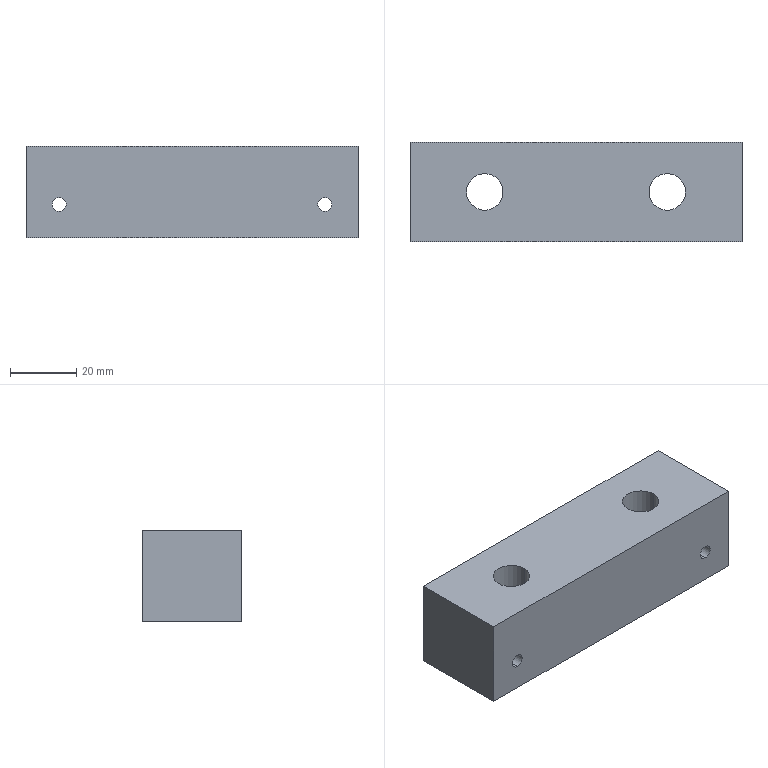Component | SolidWorks | RisingCylinderSeatPlate-1 | 1 solid | 20 faces | box 100 x 30 x 27.5 mm | volume 73803 mm3 | cylinder 12 | plane 8 | commonest cylinder face diameters 4.2 x4 17 x4 11 x4
build123d program:
from build123d import *

# Parameters (mm, degrees)
SKETCH1_W                                  = 100
SKETCH1_H                                  = 27.5
BOSS_EXTRUDE1_DEPTH                        = 30
M10_HEX_HEAD_BOLT_COUNTERBORE1_D           = 11
M10_HEX_HEAD_BOLT_COUNTERBORE1_CBORE_D     = 17
M10_HEX_HEAD_BOLT_COUNTERBORE1_CBORE_DEPTH = 10
M5_TAPPED_HOLE1_D                          = 4.2


with BuildPart() as part:
    # Sketch1 → Boss-Extrude1 (new body)
    with BuildSketch(Plane(origin=(0, 0, 0), x_dir=(1, 0, 0), z_dir=(0, 1, 0))):
        Rectangle(SKETCH1_W, SKETCH1_H)
    extrude(amount=BOSS_EXTRUDE1_DEPTH)

    # M10 Hex Head Bolt Counterbore1 (through all)
    with Locations(Plane(origin=(0, 0, -13.75), x_dir=(-1, 0, 0), z_dir=(0, 0, -1))):
        with Locations((-27.5, 15), (27.5, 15)):
            CounterBoreHole(M10_HEX_HEAD_BOLT_COUNTERBORE1_D / 2, M10_HEX_HEAD_BOLT_COUNTERBORE1_CBORE_D / 2, M10_HEX_HEAD_BOLT_COUNTERBORE1_CBORE_DEPTH)

    # M5 Tapped Hole1 (through all)
    with Locations(Plane(origin=(0, 30, 0), x_dir=(1, 0, 0), z_dir=(0, 1, 0))):
        with Locations((-40, 3.75), (40, 3.75)):
            Hole(M5_TAPPED_HOLE1_D / 2)


solid = part.part

# Placed as in the assembly
solid = solid.moved(Location((-29.507, -319.411, 406.75), (0, 0, 0)))
STEP:
#1=COLOUR_RGB('',0.7922,0.8196,0.9333);
#2=FILL_AREA_STYLE_COLOUR('',#1);
#3=FILL_AREA_STYLE('',(#2));
#4=SURFACE_STYLE_FILL_AREA(#3);
#5=SURFACE_SIDE_STYLE('',(#4));
#6=SURFACE_STYLE_USAGE(.BOTH.,#5);
#7=PRESENTATION_STYLE_ASSIGNMENT((#6));
#8=CARTESIAN_POINT('',(-2.736,-12.575,15.783));
#9=VERTEX_POINT('',#8);
#10=CARTESIAN_POINT('',(-2.736,-12.575,15.949));
#11=VERTEX_POINT('',#10);
#12=CARTESIAN_POINT('',(-2.736,-12.575,15.866));
#13=DIRECTION('',(0.,1.,0.));
#14=DIRECTION('',(0.,0.,1.));
#15=AXIS2_PLACEMENT_3D('',#12,#13,#14);
#16=CIRCLE('',#15,0.08268);
#17=EDGE_CURVE('',#9,#11,#16,.T.);
#18=ORIENTED_EDGE('',*,*,#17,.F.);
#19=CARTESIAN_POINT('',(-2.736,-11.394,15.783));
#20=VERTEX_POINT('',#19);
#21=CARTESIAN_POINT('',(-2.736,-11.394,15.783));
#22=DIRECTION('',(0.,1.,0.));
#23=VECTOR('',#22,39.37);
#24=LINE('',#21,#23);
#25=EDGE_CURVE('',#9,#20,#24,.T.);
#26=ORIENTED_EDGE('',*,*,#25,.T.);
#27=CARTESIAN_POINT('',(-2.736,-11.394,15.949));
#28=VERTEX_POINT('',#27);
#29=CARTESIAN_POINT('',(-2.736,-11.394,15.866));
#30=DIRECTION('',(0.,1.,0.));
#31=DIRECTION('',(0.,0.,1.));
#32=AXIS2_PLACEMENT_3D('',#29,#30,#31);
#33=CIRCLE('',#32,0.08268);
#34=EDGE_CURVE('',#20,#28,#33,.T.);
#35=ORIENTED_EDGE('',*,*,#34,.T.);
#36=CARTESIAN_POINT('',(-2.736,-11.394,15.949));
#37=DIRECTION('',(0.,1.,0.));
#38=VECTOR('',#37,39.37);
#39=LINE('',#36,#38);
#40=EDGE_CURVE('',#11,#28,#39,.T.);
#41=ORIENTED_EDGE('',*,*,#40,.F.);
#42=EDGE_LOOP('',(#18,#26,#35,#41));
#43=FACE_OUTER_BOUND('',#42,.T.);
#44=CARTESIAN_POINT('',(-2.736,-11.394,15.866));
#45=DIRECTION('',(0.,1.,0.));
#46=DIRECTION('',(0.,0.,1.));
#47=AXIS2_PLACEMENT_3D('',#44,#45,#46);
#48=CYLINDRICAL_SURFACE('',#47,0.08268);
#49=ADVANCED_FACE('',(#43),#48,.F.);
#50=CARTESIAN_POINT('',(0.4131,-12.575,15.783));
#51=VERTEX_POINT('',#50);
#52=CARTESIAN_POINT('',(0.4131,-12.575,15.949));
#53=VERTEX_POINT('',#52);
#54=CARTESIAN_POINT('',(0.4131,-12.575,15.866));
#55=DIRECTION('',(0.,1.,0.));
#56=DIRECTION('',(0.,0.,1.));
#57=AXIS2_PLACEMENT_3D('',#54,#55,#56);
#58=CIRCLE('',#57,0.08268);
#59=EDGE_CURVE('',#51,#53,#58,.T.);
#60=ORIENTED_EDGE('',*,*,#59,.F.);
#61=CARTESIAN_POINT('',(0.4131,-11.394,15.783));
#62=VERTEX_POINT('',#61);
#63=CARTESIAN_POINT('',(0.4131,-11.394,15.783));
#64=DIRECTION('',(0.,1.,0.));
#65=VECTOR('',#64,39.37);
#66=LINE('',#63,#65);
#67=EDGE_CURVE('',#51,#62,#66,.T.);
#68=ORIENTED_EDGE('',*,*,#67,.T.);
#69=CARTESIAN_POINT('',(0.4131,-11.394,15.949));
#70=VERTEX_POINT('',#69);
#71=CARTESIAN_POINT('',(0.4131,-11.394,15.866));
#72=DIRECTION('',(0.,1.,0.));
#73=DIRECTION('',(0.,0.,1.));
#74=AXIS2_PLACEMENT_3D('',#71,#72,#73);
#75=CIRCLE('',#74,0.08268);
#76=EDGE_CURVE('',#62,#70,#75,.T.);
#77=ORIENTED_EDGE('',*,*,#76,.T.);
#78=CARTESIAN_POINT('',(0.4131,-11.394,15.949));
#79=DIRECTION('',(0.,1.,0.));
#80=VECTOR('',#79,39.37);
#81=LINE('',#78,#80);
#82=EDGE_CURVE('',#53,#70,#81,.T.);
#83=ORIENTED_EDGE('',*,*,#82,.F.);
#84=EDGE_LOOP('',(#60,#68,#77,#83));
#85=FACE_OUTER_BOUND('',#84,.T.);
#86=CARTESIAN_POINT('',(0.4131,-11.394,15.866));
#87=DIRECTION('',(0.,1.,0.));
#88=DIRECTION('',(0.,0.,1.));
#89=AXIS2_PLACEMENT_3D('',#86,#87,#88);
#90=CYLINDRICAL_SURFACE('',#89,0.08268);
#91=ADVANCED_FACE('',(#85),#90,.F.);
#92=CARTESIAN_POINT('',(0.2556,-11.985,15.866));
#93=VERTEX_POINT('',#92);
#94=CARTESIAN_POINT('',(-0.4136,-11.985,15.866));
#95=VERTEX_POINT('',#94);
#96=CARTESIAN_POINT('',(-0.079,-11.985,15.866));
#97=DIRECTION('',(0.,0.,-1.));
#98=DIRECTION('',(-1.,0.,0.));
#99=AXIS2_PLACEMENT_3D('',#96,#97,#98);
#100=CIRCLE('',#99,0.3346);
#101=EDGE_CURVE('',#93,#95,#100,.T.);
#102=ORIENTED_EDGE('',*,*,#101,.F.);
#103=CARTESIAN_POINT('',(0.2556,-11.985,15.472));
#104=VERTEX_POINT('',#103);
#105=CARTESIAN_POINT('',(0.2556,-11.985,15.472));
#106=DIRECTION('',(0.,0.,-1.));
#107=VECTOR('',#106,39.37);
#108=LINE('',#105,#107);
#109=EDGE_CURVE('',#93,#104,#108,.T.);
#110=ORIENTED_EDGE('',*,*,#109,.T.);
#111=CARTESIAN_POINT('',(-0.4136,-11.985,15.472));
#112=VERTEX_POINT('',#111);
#113=CARTESIAN_POINT('',(-0.079,-11.985,15.472));
#114=DIRECTION('',(0.,0.,-1.));
#115=DIRECTION('',(-1.,0.,0.));
#116=AXIS2_PLACEMENT_3D('',#113,#114,#115);
#117=CIRCLE('',#116,0.3346);
#118=EDGE_CURVE('',#104,#112,#117,.T.);
#119=ORIENTED_EDGE('',*,*,#118,.T.);
#120=CARTESIAN_POINT('',(-0.4136,-11.985,15.472));
#121=DIRECTION('',(0.,0.,-1.));
#122=VECTOR('',#121,39.37);
#123=LINE('',#120,#122);
#124=EDGE_CURVE('',#95,#112,#123,.T.);
#125=ORIENTED_EDGE('',*,*,#124,.F.);
#126=EDGE_LOOP('',(#102,#110,#119,#125));
#127=FACE_OUTER_BOUND('',#126,.T.);
#128=CARTESIAN_POINT('',(-0.079,-11.985,15.472));
#129=DIRECTION('',(0.,0.,-1.));
#130=DIRECTION('',(-1.,0.,0.));
#131=AXIS2_PLACEMENT_3D('',#128,#129,#130);
#132=CYLINDRICAL_SURFACE('',#131,0.3346);
#133=ADVANCED_FACE('',(#127),#132,.F.);
#134=CARTESIAN_POINT('',(0.1375,-11.985,16.555));
#135=VERTEX_POINT('',#134);
#136=CARTESIAN_POINT('',(-0.2955,-11.985,16.555));
#137=VERTEX_POINT('',#136);
#138=CARTESIAN_POINT('',(-0.079,-11.985,16.555));
#139=DIRECTION('',(0.,0.,-1.));
#140=DIRECTION('',(-1.,0.,0.));
#141=AXIS2_PLACEMENT_3D('',#138,#139,#140);
#142=CIRCLE('',#141,0.2165);
#143=EDGE_CURVE('',#135,#137,#142,.T.);
#144=ORIENTED_EDGE('',*,*,#143,.F.);
#145=CARTESIAN_POINT('',(0.1375,-11.985,15.866));
#146=VERTEX_POINT('',#145);
#147=CARTESIAN_POINT('',(0.1375,-11.985,15.472));
#148=DIRECTION('',(0.,0.,-1.));
#149=VECTOR('',#148,39.37);
#150=LINE('',#147,#149);
#151=EDGE_CURVE('',#135,#146,#150,.T.);
#152=ORIENTED_EDGE('',*,*,#151,.T.);
#153=CARTESIAN_POINT('',(-0.2955,-11.985,15.866));
#154=VERTEX_POINT('',#153);
#155=CARTESIAN_POINT('',(-0.079,-11.985,15.866));
#156=DIRECTION('',(0.,0.,-1.));
#157=DIRECTION('',(-1.,0.,0.));
#158=AXIS2_PLACEMENT_3D('',#155,#156,#157);
#159=CIRCLE('',#158,0.2165);
#160=EDGE_CURVE('',#146,#154,#159,.T.);
#161=ORIENTED_EDGE('',*,*,#160,.T.);
#162=CARTESIAN_POINT('',(-0.2955,-11.985,15.472));
#163=DIRECTION('',(0.,0.,-1.));
#164=VECTOR('',#163,39.37);
#165=LINE('',#162,#164);
#166=EDGE_CURVE('',#137,#154,#165,.T.);
#167=ORIENTED_EDGE('',*,*,#166,.F.);
#168=EDGE_LOOP('',(#144,#152,#161,#167));
#169=FACE_OUTER_BOUND('',#168,.T.);
#170=CARTESIAN_POINT('',(-0.079,-11.985,15.472));
#171=DIRECTION('',(0.,0.,-1.));
#172=DIRECTION('',(-1.,0.,0.));
#173=AXIS2_PLACEMENT_3D('',#170,#171,#172);
#174=CYLINDRICAL_SURFACE('',#173,0.2165);
#175=ADVANCED_FACE('',(#169),#174,.F.);
#176=CARTESIAN_POINT('',(-1.91,-11.985,15.866));
#177=VERTEX_POINT('',#176);
#178=CARTESIAN_POINT('',(-2.579,-11.985,15.866));
#179=VERTEX_POINT('',#178);
#180=CARTESIAN_POINT('',(-2.244,-11.985,15.866));
#181=DIRECTION('',(0.,0.,-1.));
#182=DIRECTION('',(-1.,0.,0.));
#183=AXIS2_PLACEMENT_3D('',#180,#181,#182);
#184=CIRCLE('',#183,0.3346);
#185=EDGE_CURVE('',#177,#179,#184,.T.);
#186=ORIENTED_EDGE('',*,*,#185,.F.);
#187=CARTESIAN_POINT('',(-1.91,-11.985,15.472));
#188=VERTEX_POINT('',#187);
#189=CARTESIAN_POINT('',(-1.91,-11.985,15.472));
#190=DIRECTION('',(0.,0.,-1.));
#191=VECTOR('',#190,39.37);
#192=LINE('',#189,#191);
#193=EDGE_CURVE('',#177,#188,#192,.T.);
#194=ORIENTED_EDGE('',*,*,#193,.T.);
#195=CARTESIAN_POINT('',(-2.579,-11.985,15.472));
#196=VERTEX_POINT('',#195);
#197=CARTESIAN_POINT('',(-2.244,-11.985,15.472));
#198=DIRECTION('',(0.,0.,-1.));
#199=DIRECTION('',(-1.,0.,0.));
#200=AXIS2_PLACEMENT_3D('',#197,#198,#199);
#201=CIRCLE('',#200,0.3346);
#202=EDGE_CURVE('',#188,#196,#201,.T.);
#203=ORIENTED_EDGE('',*,*,#202,.T.);
#204=CARTESIAN_POINT('',(-2.579,-11.985,15.472));
#205=DIRECTION('',(0.,0.,-1.));
#206=VECTOR('',#205,39.37);
#207=LINE('',#204,#206);
#208=EDGE_CURVE('',#179,#196,#207,.T.);
#209=ORIENTED_EDGE('',*,*,#208,.F.);
#210=EDGE_LOOP('',(#186,#194,#203,#209));
#211=FACE_OUTER_BOUND('',#210,.T.);
#212=CARTESIAN_POINT('',(-2.244,-11.985,15.472));
#213=DIRECTION('',(0.,0.,-1.));
#214=DIRECTION('',(-1.,0.,0.));
#215=AXIS2_PLACEMENT_3D('',#212,#213,#214);
#216=CYLINDRICAL_SURFACE('',#215,0.3346);
#217=ADVANCED_FACE('',(#211),#216,.F.);
#218=CARTESIAN_POINT('',(-2.028,-11.985,16.555));
#219=VERTEX_POINT('',#218);
#220=CARTESIAN_POINT('',(-2.461,-11.985,16.555));
#221=VERTEX_POINT('',#220);
#222=CARTESIAN_POINT('',(-2.244,-11.985,16.555));
#223=DIRECTION('',(0.,0.,-1.));
#224=DIRECTION('',(-1.,0.,0.));
#225=AXIS2_PLACEMENT_3D('',#222,#223,#224);
#226=CIRCLE('',#225,0.2165);
#227=EDGE_CURVE('',#219,#221,#226,.T.);
#228=ORIENTED_EDGE('',*,*,#227,.F.);
#229=CARTESIAN_POINT('',(-2.028,-11.985,15.866));
#230=VERTEX_POINT('',#229);
#231=CARTESIAN_POINT('',(-2.028,-11.985,15.472));
#232=DIRECTION('',(0.,0.,-1.));
#233=VECTOR('',#232,39.37);
#234=LINE('',#231,#233);
#235=EDGE_CURVE('',#219,#230,#234,.T.);
#236=ORIENTED_EDGE('',*,*,#235,.T.);
#237=CARTESIAN_POINT('',(-2.461,-11.985,15.866));
#238=VERTEX_POINT('',#237);
#239=CARTESIAN_POINT('',(-2.244,-11.985,15.866));
#240=DIRECTION('',(0.,0.,-1.));
#241=DIRECTION('',(-1.,0.,0.));
#242=AXIS2_PLACEMENT_3D('',#239,#240,#241);
#243=CIRCLE('',#242,0.2165);
#244=EDGE_CURVE('',#230,#238,#243,.T.);
#245=ORIENTED_EDGE('',*,*,#244,.T.);
#246=CARTESIAN_POINT('',(-2.461,-11.985,15.472));
#247=DIRECTION('',(0.,0.,-1.));
#248=VECTOR('',#247,39.37);
#249=LINE('',#246,#248);
#250=EDGE_CURVE('',#221,#238,#249,.T.);
#251=ORIENTED_EDGE('',*,*,#250,.F.);
#252=EDGE_LOOP('',(#228,#236,#245,#251));
#253=FACE_OUTER_BOUND('',#252,.T.);
#254=CARTESIAN_POINT('',(-2.244,-11.985,15.472));
#255=DIRECTION('',(0.,0.,-1.));
#256=DIRECTION('',(-1.,0.,0.));
#257=AXIS2_PLACEMENT_3D('',#254,#255,#256);
#258=CYLINDRICAL_SURFACE('',#257,0.2165);
#259=ADVANCED_FACE('',(#253),#258,.F.);
#260=CARTESIAN_POINT('',(-3.13,-12.575,15.472));
#261=VERTEX_POINT('',#260);
#262=CARTESIAN_POINT('',(-3.13,-12.575,16.555));
#263=VERTEX_POINT('',#262);
#264=CARTESIAN_POINT('',(-3.13,-12.575,16.555));
#265=DIRECTION('',(0.,0.,1.));
#266=VECTOR('',#265,39.37);
#267=LINE('',#264,#266);
#268=EDGE_CURVE('',#261,#263,#267,.T.);
#269=ORIENTED_EDGE('',*,*,#268,.T.);
#270=CARTESIAN_POINT('',(-3.13,-11.394,16.555));
#271=VERTEX_POINT('',#270);
#272=CARTESIAN_POINT('',(-3.13,-11.394,16.555));
#273=DIRECTION('',(0.,-1.,0.));
#274=VECTOR('',#273,39.37);
#275=LINE('',#272,#274);
#276=EDGE_CURVE('',#271,#263,#275,.T.);
#277=ORIENTED_EDGE('',*,*,#276,.F.);
#278=CARTESIAN_POINT('',(-3.13,-11.394,15.472));
#279=VERTEX_POINT('',#278);
#280=CARTESIAN_POINT('',(-3.13,-11.394,16.555));
#281=DIRECTION('',(0.,0.,1.));
#282=VECTOR('',#281,39.37);
#283=LINE('',#280,#282);
#284=EDGE_CURVE('',#279,#271,#283,.T.);
#285=ORIENTED_EDGE('',*,*,#284,.F.);
#286=CARTESIAN_POINT('',(-3.13,-11.394,15.472));
#287=DIRECTION('',(0.,-1.,0.));
#288=VECTOR('',#287,39.37);
#289=LINE('',#286,#288);
#290=EDGE_CURVE('',#279,#261,#289,.T.);
#291=ORIENTED_EDGE('',*,*,#290,.T.);
#292=EDGE_LOOP('',(#269,#277,#285,#291));
#293=FACE_OUTER_BOUND('',#292,.T.);
#294=CARTESIAN_POINT('',(-3.13,-11.394,16.555));
#295=DIRECTION('',(1.,0.,0.));
#296=DIRECTION('',(0.,0.,-1.));
#297=AXIS2_PLACEMENT_3D('',#294,#295,#296);
#298=PLANE('',#297);
#299=ADVANCED_FACE('',(#293),#298,.F.);
#300=CARTESIAN_POINT('',(-0.079,-11.985,16.555));
#301=DIRECTION('',(0.,0.,-1.));
#302=DIRECTION('',(-1.,0.,0.));
#303=AXIS2_PLACEMENT_3D('',#300,#301,#302);
#304=CIRCLE('',#303,0.2165);
#305=EDGE_CURVE('',#137,#135,#304,.T.);
#306=ORIENTED_EDGE('',*,*,#305,.T.);
#307=ORIENTED_EDGE('',*,*,#143,.T.);
#308=EDGE_LOOP('',(#306,#307));
#309=FACE_BOUND('',#308,.T.);
#310=CARTESIAN_POINT('',(-2.244,-11.985,16.555));
#311=DIRECTION('',(0.,0.,-1.));
#312=DIRECTION('',(-1.,0.,0.));
#313=AXIS2_PLACEMENT_3D('',#310,#311,#312);
#314=CIRCLE('',#313,0.2165);
#315=EDGE_CURVE('',#221,#219,#314,.T.);
#316=ORIENTED_EDGE('',*,*,#315,.T.);
#317=ORIENTED_EDGE('',*,*,#227,.T.);
#318=EDGE_LOOP('',(#316,#317));
#319=FACE_BOUND('',#318,.T.);
#320=CARTESIAN_POINT('',(0.8068,-12.575,16.555));
#321=VERTEX_POINT('',#320);
#322=CARTESIAN_POINT('',(0.8068,-12.575,16.555));
#323=DIRECTION('',(1.,0.,-0.));
#324=VECTOR('',#323,39.37);
#325=LINE('',#322,#324);
#326=EDGE_CURVE('',#263,#321,#325,.T.);
#327=ORIENTED_EDGE('',*,*,#326,.T.);
#328=CARTESIAN_POINT('',(0.8068,-11.394,16.555));
#329=VERTEX_POINT('',#328);
#330=CARTESIAN_POINT('',(0.8068,-11.394,16.555));
#331=DIRECTION('',(0.,-1.,0.));
#332=VECTOR('',#331,39.37);
#333=LINE('',#330,#332);
#334=EDGE_CURVE('',#329,#321,#333,.T.);
#335=ORIENTED_EDGE('',*,*,#334,.F.);
#336=CARTESIAN_POINT('',(0.8068,-11.394,16.555));
#337=DIRECTION('',(1.,0.,-0.));
#338=VECTOR('',#337,39.37);
#339=LINE('',#336,#338);
#340=EDGE_CURVE('',#271,#329,#339,.T.);
#341=ORIENTED_EDGE('',*,*,#340,.F.);
#342=ORIENTED_EDGE('',*,*,#276,.T.);
#343=EDGE_LOOP('',(#327,#335,#341,#342));
#344=FACE_OUTER_BOUND('',#343,.T.);
#345=CARTESIAN_POINT('',(0.8068,-11.394,16.555));
#346=DIRECTION('',(-0.,0.,-1.));
#347=DIRECTION('',(-1.,0.,0.));
#348=AXIS2_PLACEMENT_3D('',#345,#346,#347);
#349=PLANE('',#348);
#350=ADVANCED_FACE('',(#309,#319,#344),#349,.F.);
#351=CARTESIAN_POINT('',(0.8068,-12.575,15.472));
#352=VERTEX_POINT('',#351);
#353=CARTESIAN_POINT('',(0.8068,-12.575,16.555));
#354=DIRECTION('',(0.,0.,-1.));
#355=VECTOR('',#354,39.37);
#356=LINE('',#353,#355);
#357=EDGE_CURVE('',#321,#352,#356,.T.);
#358=ORIENTED_EDGE('',*,*,#357,.T.);
#359=CARTESIAN_POINT('',(0.8068,-11.394,15.472));
#360=VERTEX_POINT('',#359);
#361=CARTESIAN_POINT('',(0.8068,-11.394,15.472));
#362=DIRECTION('',(0.,-1.,0.));
#363=VECTOR('',#362,39.37);
#364=LINE('',#361,#363);
#365=EDGE_CURVE('',#360,#352,#364,.T.);
#366=ORIENTED_EDGE('',*,*,#365,.F.);
#367=CARTESIAN_POINT('',(0.8068,-11.394,16.555));
#368=DIRECTION('',(0.,0.,-1.));
#369=VECTOR('',#368,39.37);
#370=LINE('',#367,#369);
#371=EDGE_CURVE('',#329,#360,#370,.T.);
#372=ORIENTED_EDGE('',*,*,#371,.F.);
#373=ORIENTED_EDGE('',*,*,#334,.T.);
#374=EDGE_LOOP('',(#358,#366,#372,#373));
#375=FACE_OUTER_BOUND('',#374,.T.);
#376=CARTESIAN_POINT('',(0.8068,-11.394,16.555));
#377=DIRECTION('',(-1.,0.,0.));
#378=DIRECTION('',(0.,0.,1.));
#379=AXIS2_PLACEMENT_3D('',#376,#377,#378);
#380=PLANE('',#379);
#381=ADVANCED_FACE('',(#375),#380,.F.);
#382=CARTESIAN_POINT('',(-0.079,-11.985,15.472));
#383=DIRECTION('',(0.,0.,-1.));
#384=DIRECTION('',(-1.,0.,0.));
#385=AXIS2_PLACEMENT_3D('',#382,#383,#384);
#386=CIRCLE('',#385,0.3346);
#387=EDGE_CURVE('',#112,#104,#386,.T.);
#388=ORIENTED_EDGE('',*,*,#387,.F.);
#389=ORIENTED_EDGE('',*,*,#118,.F.);
#390=EDGE_LOOP('',(#388,#389));
#391=FACE_BOUND('',#390,.T.);
#392=CARTESIAN_POINT('',(-2.244,-11.985,15.472));
#393=DIRECTION('',(0.,0.,-1.));
#394=DIRECTION('',(-1.,0.,0.));
#395=AXIS2_PLACEMENT_3D('',#392,#393,#394);
#396=CIRCLE('',#395,0.3346);
#397=EDGE_CURVE('',#196,#188,#396,.T.);
#398=ORIENTED_EDGE('',*,*,#397,.F.);
#399=ORIENTED_EDGE('',*,*,#202,.F.);
#400=EDGE_LOOP('',(#398,#399));
#401=FACE_BOUND('',#400,.T.);
#402=CARTESIAN_POINT('',(0.8068,-12.575,15.472));
#403=DIRECTION('',(-1.,0.,0.));
#404=VECTOR('',#403,39.37);
#405=LINE('',#402,#404);
#406=EDGE_CURVE('',#352,#261,#405,.T.);
#407=ORIENTED_EDGE('',*,*,#406,.T.);
#408=ORIENTED_EDGE('',*,*,#290,.F.);
#409=CARTESIAN_POINT('',(0.8068,-11.394,15.472));
#410=DIRECTION('',(-1.,0.,0.));
#411=VECTOR('',#410,39.37);
#412=LINE('',#409,#411);
#413=EDGE_CURVE('',#360,#279,#412,.T.);
#414=ORIENTED_EDGE('',*,*,#413,.F.);
#415=ORIENTED_EDGE('',*,*,#365,.T.);
#416=EDGE_LOOP('',(#407,#408,#414,#415));
#417=FACE_OUTER_BOUND('',#416,.T.);
#418=CARTESIAN_POINT('',(0.8068,-11.394,15.472));
#419=DIRECTION('',(0.,0.,1.));
#420=DIRECTION('',(1.,0.,-0.));
#421=AXIS2_PLACEMENT_3D('',#418,#419,#420);
#422=PLANE('',#421);
#423=ADVANCED_FACE('',(#391,#401,#417),#422,.F.);
#424=CARTESIAN_POINT('',(-2.736,-11.394,15.866));
#425=DIRECTION('',(0.,1.,0.));
#426=DIRECTION('',(0.,0.,1.));
#427=AXIS2_PLACEMENT_3D('',#424,#425,#426);
#428=CIRCLE('',#427,0.08268);
#429=EDGE_CURVE('',#28,#20,#428,.T.);
#430=ORIENTED_EDGE('',*,*,#429,.F.);
#431=ORIENTED_EDGE('',*,*,#34,.F.);
#432=EDGE_LOOP('',(#430,#431));
#433=FACE_BOUND('',#432,.T.);
#434=CARTESIAN_POINT('',(0.4131,-11.394,15.866));
#435=DIRECTION('',(0.,1.,0.));
#436=DIRECTION('',(0.,0.,1.));
#437=AXIS2_PLACEMENT_3D('',#434,#435,#436);
#438=CIRCLE('',#437,0.08268);
#439=EDGE_CURVE('',#70,#62,#438,.T.);
#440=ORIENTED_EDGE('',*,*,#439,.F.);
#441=ORIENTED_EDGE('',*,*,#76,.F.);
#442=EDGE_LOOP('',(#440,#441));
#443=FACE_BOUND('',#442,.T.);
#444=ORIENTED_EDGE('',*,*,#284,.T.);
#445=ORIENTED_EDGE('',*,*,#340,.T.);
#446=ORIENTED_EDGE('',*,*,#371,.T.);
#447=ORIENTED_EDGE('',*,*,#413,.T.);
#448=EDGE_LOOP('',(#444,#445,#446,#447));
#449=FACE_OUTER_BOUND('',#448,.T.);
#450=CARTESIAN_POINT('',(-1.162,-11.394,16.014));
#451=DIRECTION('',(0.,1.,0.));
#452=DIRECTION('',(0.,0.,1.));
#453=AXIS2_PLACEMENT_3D('',#450,#451,#452);
#454=PLANE('',#453);
#455=ADVANCED_FACE('',(#433,#443,#449),#454,.T.);
#456=CARTESIAN_POINT('',(-2.736,-12.575,15.866));
#457=DIRECTION('',(0.,1.,0.));
#458=DIRECTION('',(0.,0.,1.));
#459=AXIS2_PLACEMENT_3D('',#456,#457,#458);
#460=CIRCLE('',#459,0.08268);
#461=EDGE_CURVE('',#11,#9,#460,.T.);
#462=ORIENTED_EDGE('',*,*,#461,.T.);
#463=ORIENTED_EDGE('',*,*,#17,.T.);
#464=EDGE_LOOP('',(#462,#463));
#465=FACE_BOUND('',#464,.T.);
#466=CARTESIAN_POINT('',(0.4131,-12.575,15.866));
#467=DIRECTION('',(0.,1.,0.));
#468=DIRECTION('',(0.,0.,1.));
#469=AXIS2_PLACEMENT_3D('',#466,#467,#468);
#470=CIRCLE('',#469,0.08268);
#471=EDGE_CURVE('',#53,#51,#470,.T.);
#472=ORIENTED_EDGE('',*,*,#471,.T.);
#473=ORIENTED_EDGE('',*,*,#59,.T.);
#474=EDGE_LOOP('',(#472,#473));
#475=FACE_BOUND('',#474,.T.);
#476=ORIENTED_EDGE('',*,*,#268,.F.);
#477=ORIENTED_EDGE('',*,*,#406,.F.);
#478=ORIENTED_EDGE('',*,*,#357,.F.);
#479=ORIENTED_EDGE('',*,*,#326,.F.);
#480=EDGE_LOOP('',(#476,#477,#478,#479));
#481=FACE_OUTER_BOUND('',#480,.T.);
#482=CARTESIAN_POINT('',(-1.162,-12.575,16.014));
#483=DIRECTION('',(0.,1.,0.));
#484=DIRECTION('',(0.,0.,1.));
#485=AXIS2_PLACEMENT_3D('',#482,#483,#484);
#486=PLANE('',#485);
#487=ADVANCED_FACE('',(#465,#475,#481),#486,.F.);
#488=ORIENTED_EDGE('',*,*,#235,.F.);
#489=ORIENTED_EDGE('',*,*,#315,.F.);
#490=ORIENTED_EDGE('',*,*,#250,.T.);
#491=CARTESIAN_POINT('',(-2.244,-11.985,15.866));
#492=DIRECTION('',(0.,0.,-1.));
#493=DIRECTION('',(-1.,0.,0.));
#494=AXIS2_PLACEMENT_3D('',#491,#492,#493);
#495=CIRCLE('',#494,0.2165);
#496=EDGE_CURVE('',#238,#230,#495,.T.);
#497=ORIENTED_EDGE('',*,*,#496,.T.);
#498=EDGE_LOOP('',(#488,#489,#490,#497));
#499=FACE_OUTER_BOUND('',#498,.T.);
#500=CARTESIAN_POINT('',(-2.244,-11.985,15.472));
#501=DIRECTION('',(0.,0.,-1.));
#502=DIRECTION('',(-1.,0.,0.));
#503=AXIS2_PLACEMENT_3D('',#500,#501,#502);
#504=CYLINDRICAL_SURFACE('',#503,0.2165);
#505=ADVANCED_FACE('',(#499),#504,.F.);
#506=ORIENTED_EDGE('',*,*,#496,.F.);
#507=ORIENTED_EDGE('',*,*,#244,.F.);
#508=EDGE_LOOP('',(#506,#507));
#509=FACE_BOUND('',#508,.T.);
#510=CARTESIAN_POINT('',(-2.244,-11.985,15.866));
#511=DIRECTION('',(0.,0.,-1.));
#512=DIRECTION('',(-1.,0.,0.));
#513=AXIS2_PLACEMENT_3D('',#510,#511,#512);
#514=CIRCLE('',#513,0.3346);
#515=EDGE_CURVE('',#179,#177,#514,.T.);
#516=ORIENTED_EDGE('',*,*,#515,.T.);
#517=ORIENTED_EDGE('',*,*,#185,.T.);
#518=EDGE_LOOP('',(#516,#517));
#519=FACE_OUTER_BOUND('',#518,.T.);
#520=CARTESIAN_POINT('',(-2.028,-11.985,15.866));
#521=DIRECTION('',(0.,0.,1.));
#522=DIRECTION('',(1.,0.,0.));
#523=AXIS2_PLACEMENT_3D('',#520,#521,#522);
#524=PLANE('',#523);
#525=ADVANCED_FACE('',(#509,#519),#524,.F.);
#526=ORIENTED_EDGE('',*,*,#193,.F.);
#527=ORIENTED_EDGE('',*,*,#515,.F.);
#528=ORIENTED_EDGE('',*,*,#208,.T.);
#529=ORIENTED_EDGE('',*,*,#397,.T.);
#530=EDGE_LOOP('',(#526,#527,#528,#529));
#531=FACE_OUTER_BOUND('',#530,.T.);
#532=CARTESIAN_POINT('',(-2.244,-11.985,15.472));
#533=DIRECTION('',(0.,0.,-1.));
#534=DIRECTION('',(-1.,0.,0.));
#535=AXIS2_PLACEMENT_3D('',#532,#533,#534);
#536=CYLINDRICAL_SURFACE('',#535,0.3346);
#537=ADVANCED_FACE('',(#531),#536,.F.);
#538=ORIENTED_EDGE('',*,*,#151,.F.);
#539=ORIENTED_EDGE('',*,*,#305,.F.);
#540=ORIENTED_EDGE('',*,*,#166,.T.);
#541=CARTESIAN_POINT('',(-0.079,-11.985,15.866));
#542=DIRECTION('',(0.,0.,-1.));
#543=DIRECTION('',(-1.,0.,0.));
#544=AXIS2_PLACEMENT_3D('',#541,#542,#543);
#545=CIRCLE('',#544,0.2165);
#546=EDGE_CURVE('',#154,#146,#545,.T.);
#547=ORIENTED_EDGE('',*,*,#546,.T.);
#548=EDGE_LOOP('',(#538,#539,#540,#547));
#549=FACE_OUTER_BOUND('',#548,.T.);
#550=CARTESIAN_POINT('',(-0.079,-11.985,15.472));
#551=DIRECTION('',(0.,0.,-1.));
#552=DIRECTION('',(-1.,0.,0.));
#553=AXIS2_PLACEMENT_3D('',#550,#551,#552);
#554=CYLINDRICAL_SURFACE('',#553,0.2165);
#555=ADVANCED_FACE('',(#549),#554,.F.);
#556=ORIENTED_EDGE('',*,*,#546,.F.);
#557=ORIENTED_EDGE('',*,*,#160,.F.);
#558=EDGE_LOOP('',(#556,#557));
#559=FACE_BOUND('',#558,.T.);
#560=CARTESIAN_POINT('',(-0.079,-11.985,15.866));
#561=DIRECTION('',(0.,0.,-1.));
#562=DIRECTION('',(-1.,0.,0.));
#563=AXIS2_PLACEMENT_3D('',#560,#561,#562);
#564=CIRCLE('',#563,0.3346);
#565=EDGE_CURVE('',#95,#93,#564,.T.);
#566=ORIENTED_EDGE('',*,*,#565,.T.);
#567=ORIENTED_EDGE('',*,*,#101,.T.);
#568=EDGE_LOOP('',(#566,#567));
#569=FACE_OUTER_BOUND('',#568,.T.);
#570=CARTESIAN_POINT('',(0.1375,-11.985,15.866));
#571=DIRECTION('',(0.,0.,1.));
#572=DIRECTION('',(1.,0.,0.));
#573=AXIS2_PLACEMENT_3D('',#570,#571,#572);
#574=PLANE('',#573);
#575=ADVANCED_FACE('',(#559,#569),#574,.F.);
#576=ORIENTED_EDGE('',*,*,#109,.F.);
#577=ORIENTED_EDGE('',*,*,#565,.F.);
#578=ORIENTED_EDGE('',*,*,#124,.T.);
#579=ORIENTED_EDGE('',*,*,#387,.T.);
#580=EDGE_LOOP('',(#576,#577,#578,#579));
#581=FACE_OUTER_BOUND('',#580,.T.);
#582=CARTESIAN_POINT('',(-0.079,-11.985,15.472));
#583=DIRECTION('',(0.,0.,-1.));
#584=DIRECTION('',(-1.,0.,0.));
#585=AXIS2_PLACEMENT_3D('',#582,#583,#584);
#586=CYLINDRICAL_SURFACE('',#585,0.3346);
#587=ADVANCED_FACE('',(#581),#586,.F.);
#588=ORIENTED_EDGE('',*,*,#67,.F.);
#589=ORIENTED_EDGE('',*,*,#471,.F.);
#590=ORIENTED_EDGE('',*,*,#82,.T.);
#591=ORIENTED_EDGE('',*,*,#439,.T.);
#592=EDGE_LOOP('',(#588,#589,#590,#591));
#593=FACE_OUTER_BOUND('',#592,.T.);
#594=CARTESIAN_POINT('',(0.4131,-11.394,15.866));
#595=DIRECTION('',(0.,1.,0.));
#596=DIRECTION('',(0.,0.,1.));
#597=AXIS2_PLACEMENT_3D('',#594,#595,#596);
#598=CYLINDRICAL_SURFACE('',#597,0.08268);
#599=ADVANCED_FACE('',(#593),#598,.F.);
#600=ORIENTED_EDGE('',*,*,#25,.F.);
#601=ORIENTED_EDGE('',*,*,#461,.F.);
#602=ORIENTED_EDGE('',*,*,#40,.T.);
#603=ORIENTED_EDGE('',*,*,#429,.T.);
#604=EDGE_LOOP('',(#600,#601,#602,#603));
#605=FACE_OUTER_BOUND('',#604,.T.);
#606=CARTESIAN_POINT('',(-2.736,-11.394,15.866));
#607=DIRECTION('',(0.,1.,0.));
#608=DIRECTION('',(0.,0.,1.));
#609=AXIS2_PLACEMENT_3D('',#606,#607,#608);
#610=CYLINDRICAL_SURFACE('',#609,0.08268);
#611=ADVANCED_FACE('',(#605),#610,.F.);
#612=CLOSED_SHELL('',(#49,#91,#133,#175,#217,#259,#299,#350,#381,#423,#455,#487,#505,#525,#537,#555,#575,#587,#599,#611));
#613=MANIFOLD_SOLID_BREP('',#612);
#614=STYLED_ITEM('',(#7),#613);
#615=(LENGTH_UNIT()NAMED_UNIT(*)SI_UNIT($,.METRE.));
#616=LENGTH_MEASURE_WITH_UNIT(LENGTH_MEASURE(0.0254),#615);
#617=DIMENSIONAL_EXPONENTS(1.,0.,0.,0.,0.,0.,0.);
#618=(CONVERSION_BASED_UNIT('',#616)LENGTH_UNIT()NAMED_UNIT(#617));
#619=UNCERTAINTY_MEASURE_WITH_UNIT(LENGTH_MEASURE(0.00001),#618,'','');
#620=(NAMED_UNIT(*)PLANE_ANGLE_UNIT()SI_UNIT($,.RADIAN.));
#621=(NAMED_UNIT(*)SI_UNIT($,.STERADIAN.)SOLID_ANGLE_UNIT());
#622=(GEOMETRIC_REPRESENTATION_CONTEXT(3)GLOBAL_UNCERTAINTY_ASSIGNED_CONTEXT((#619))GLOBAL_UNIT_ASSIGNED_CONTEXT((#618,#620,#621))REPRESENTATION_CONTEXT('',''));
#623=MECHANICAL_DESIGN_GEOMETRIC_PRESENTATION_REPRESENTATION('',(#614),#622);
#624=PRESENTATION_LAYER_ASSIGNMENT('','',(#614));
#625=CARTESIAN_POINT('',(0.,0.,0.));
#626=DIRECTION('',(0.,0.,1.));
#627=DIRECTION('',(1.,0.,0.));
#628=AXIS2_PLACEMENT_3D('',#625,#626,#627);
#629=(LENGTH_UNIT()NAMED_UNIT(*)SI_UNIT($,.METRE.));
#630=LENGTH_MEASURE_WITH_UNIT(LENGTH_MEASURE(0.0254),#629);
#631=DIMENSIONAL_EXPONENTS(1.,0.,0.,0.,0.,0.,0.);
#632=(CONVERSION_BASED_UNIT('',#630)LENGTH_UNIT()NAMED_UNIT(#631));
#633=UNCERTAINTY_MEASURE_WITH_UNIT(LENGTH_MEASURE(0.00001),#632,'','');
#634=(NAMED_UNIT(*)PLANE_ANGLE_UNIT()SI_UNIT($,.RADIAN.));
#635=(NAMED_UNIT(*)SI_UNIT($,.STERADIAN.)SOLID_ANGLE_UNIT());
#636=(GEOMETRIC_REPRESENTATION_CONTEXT(3)GLOBAL_UNCERTAINTY_ASSIGNED_CONTEXT((#633))GLOBAL_UNIT_ASSIGNED_CONTEXT((#632,#634,#635))REPRESENTATION_CONTEXT('',''));
#637=ADVANCED_BREP_SHAPE_REPRESENTATION('',(#613,#628),#636);